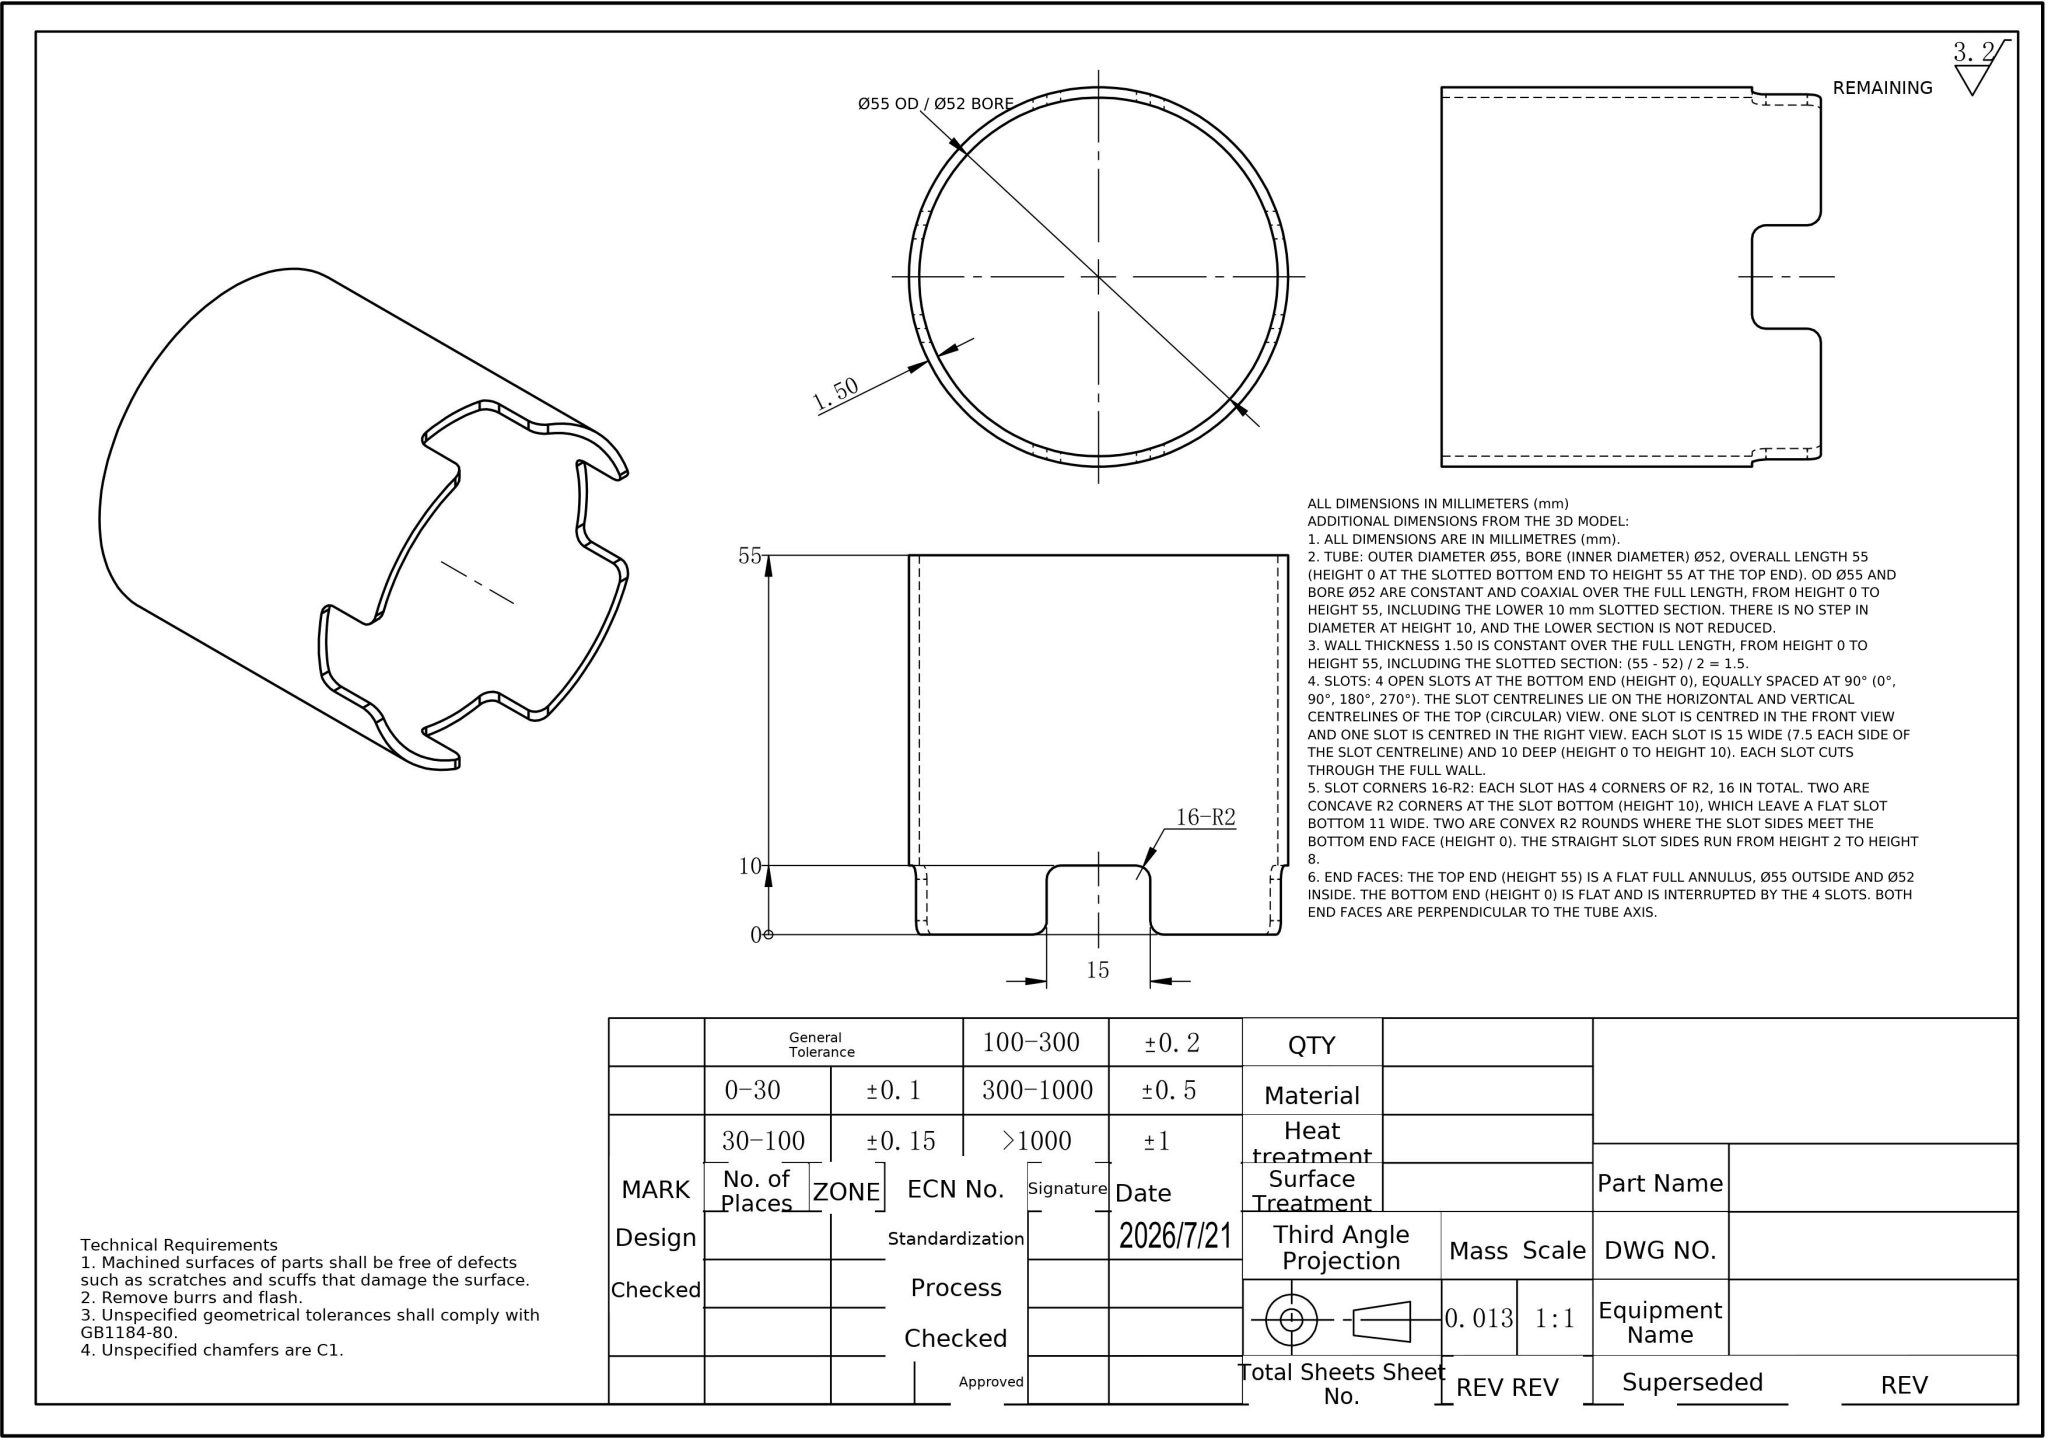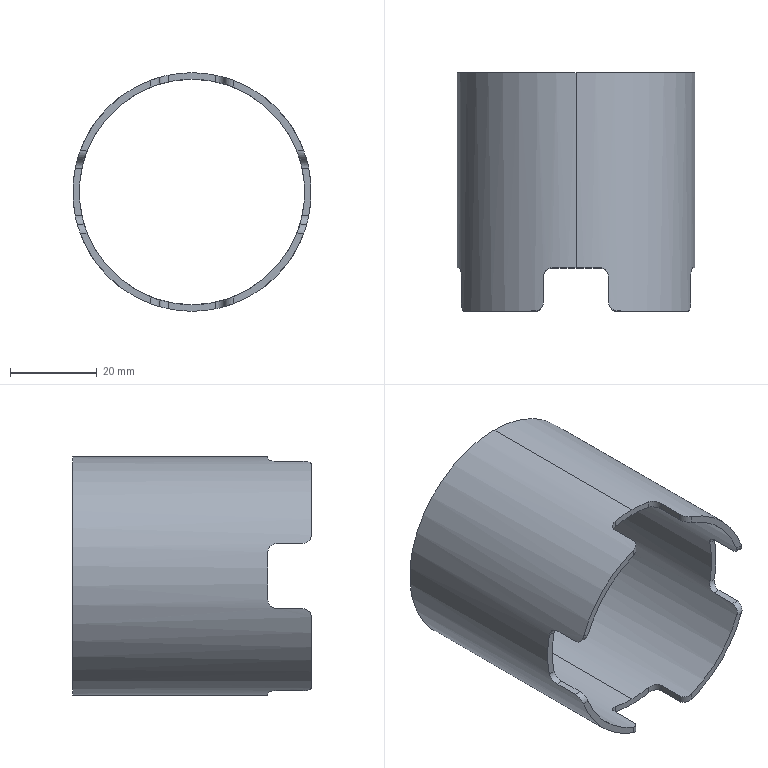Part | NX | mm | 1 solid | 37 faces | box 55 x 55 x 55 mm | volume 12954 mm3 | cylinder 20 | plane 17 | commonest cylinder face diameters 4 x16 52 x2 55 x2